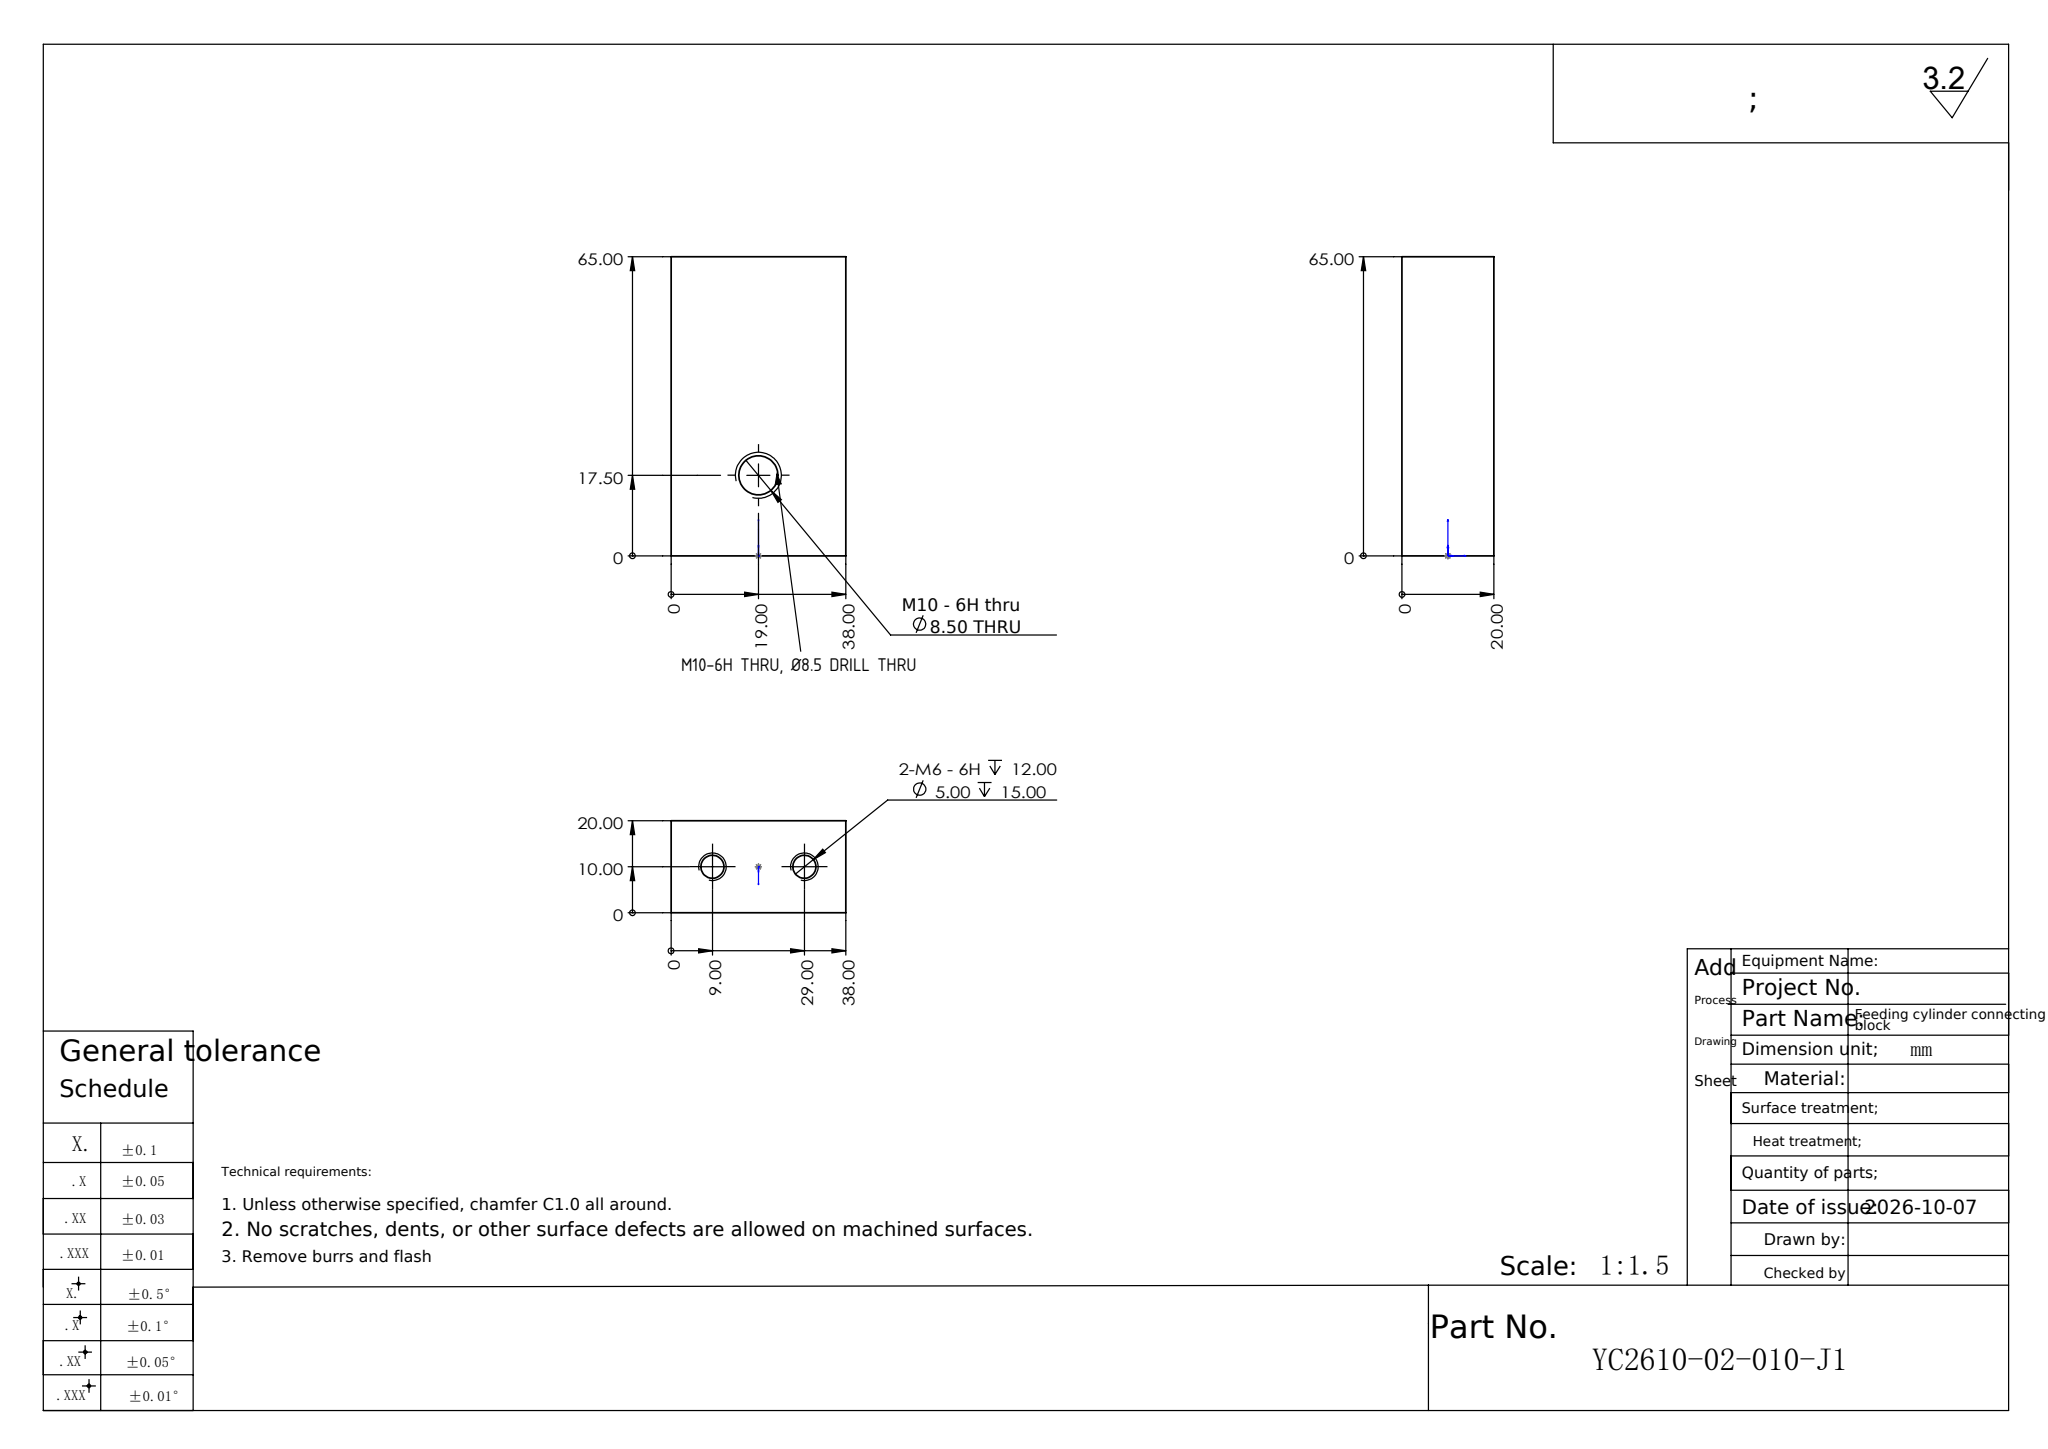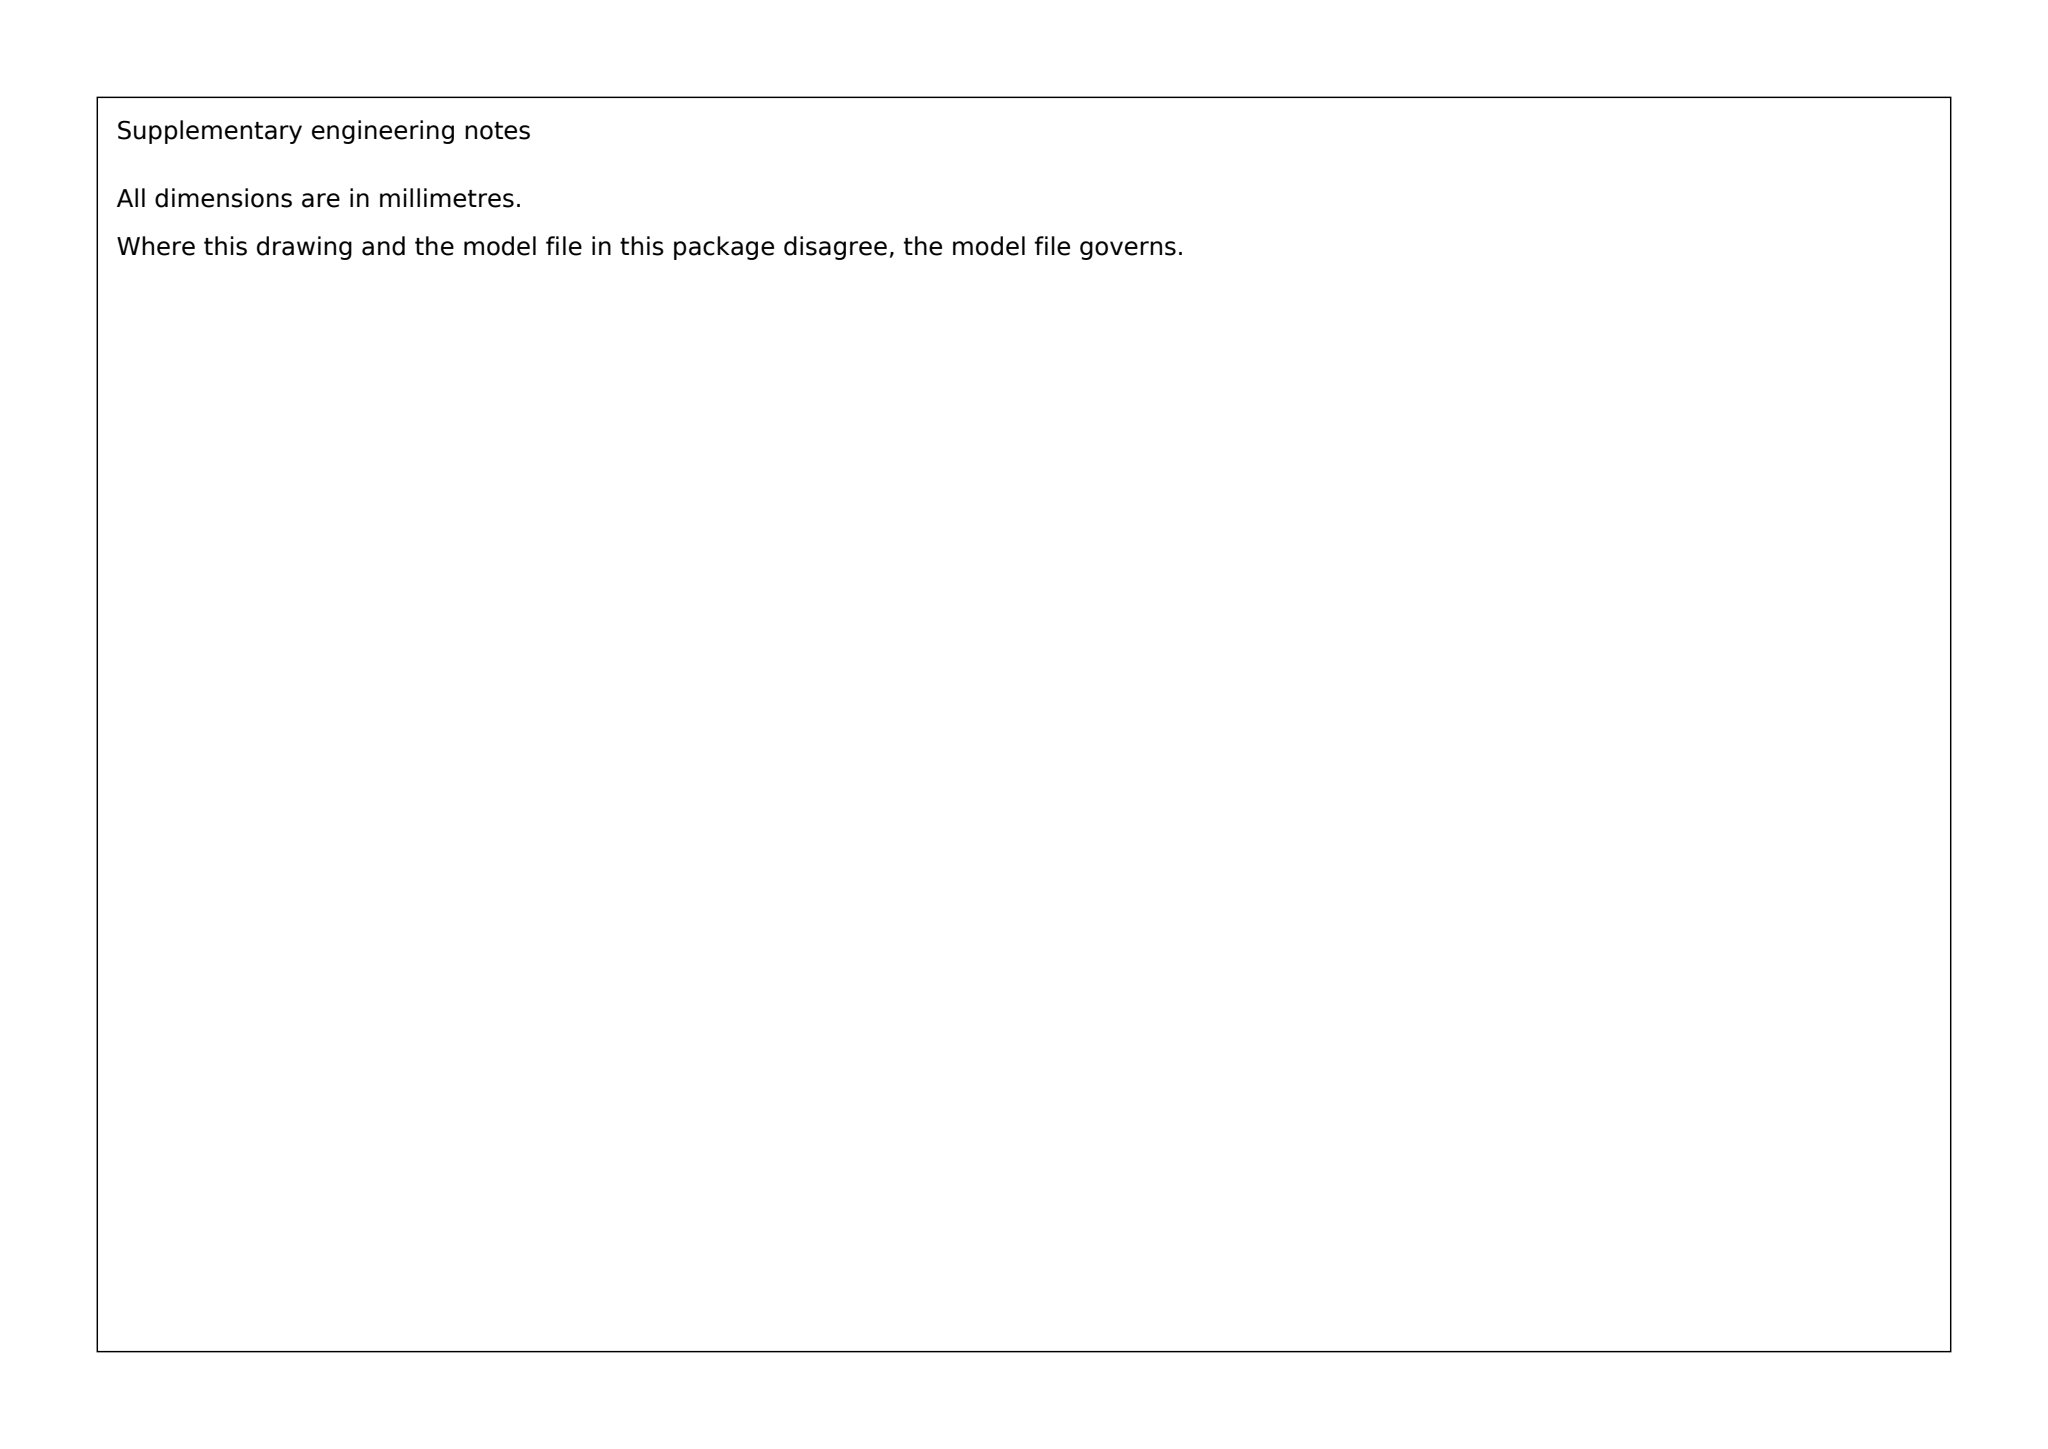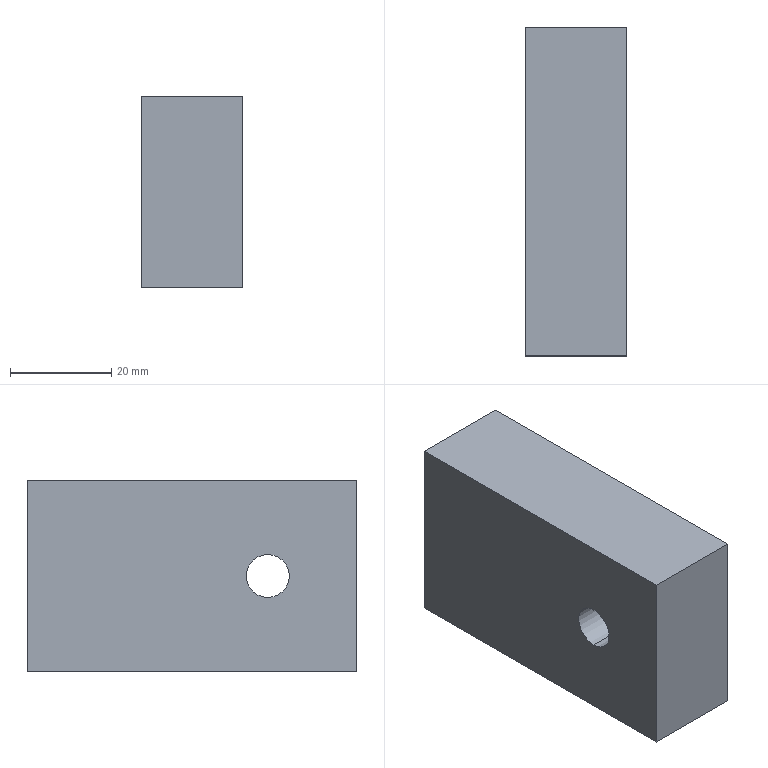Part | SolidWorks | mm | 1 solid | 16 faces | box 20 x 65 x 38 mm | volume 47656 mm3 | cylinder 6 | plane 6 | cone 4 | commonest cylinder face diameters 5 x4 8.5 x2
Drawing notes:
M10-6H THRU, Ø8.5 DRILL THRU 20 THK | from the solid: cylinder dia 8.5 axis x, length 20.0 = full x extent (planes x=0, x=20)
build123d program:
from build123d import *

# Parameters (mm, degrees)
SKETCH1_W             = 20
SKETCH1_H             = 38
BOSS_EXTRUDE1_DEPTH   = 65
M6_TAPPED_HOLE1_D     = 5
M6_TAPPED_HOLE1_DEPTH = 15
M6_TAPPED_HOLE1_TIP   = 1.502
M10_TAPPED_HOLE1_D    = 8.5


with BuildPart() as part:
    # Sketch1 → Boss-Extrude1 (new body)
    with BuildSketch(Plane(origin=(0, 0, 0), x_dir=(1, 0, 0), z_dir=(0, 1, 0))):
        Rectangle(SKETCH1_W, SKETCH1_H)
    extrude(amount=BOSS_EXTRUDE1_DEPTH)

    # M6 Tapped Hole1
    with Locations(Plane(origin=(0, 65, 0), x_dir=(1, 0, 0), z_dir=(0, 1, 0))):
        with Locations((0, 10), (0, -10)):
            Hole(M6_TAPPED_HOLE1_D / 2, depth=M6_TAPPED_HOLE1_DEPTH)
            with Locations((0, 0, -(M6_TAPPED_HOLE1_DEPTH + M6_TAPPED_HOLE1_TIP / 2))):  # 118° drill point
                Cone(0, M6_TAPPED_HOLE1_D / 2, M6_TAPPED_HOLE1_TIP, mode=Mode.SUBTRACT)

    # M10 Tapped Hole1 (through all)
    with Locations(Plane(origin=(10, 0, 0), x_dir=(0, 0, -1), z_dir=(1, 0, 0))):
        with Locations((0, 17.5)):
            Hole(M10_TAPPED_HOLE1_D / 2)


solid = part.part
STEP:
#1=CARTESIAN_POINT('',(-10.,17.5,4.25));
#2=VERTEX_POINT('',#1);
#3=CARTESIAN_POINT('',(-10.,17.5,-4.25));
#4=VERTEX_POINT('',#3);
#5=CARTESIAN_POINT('',(-10.,17.5,0.));
#6=DIRECTION('',(1.,0.,-0.));
#7=DIRECTION('',(0.,0.,-1.));
#8=AXIS2_PLACEMENT_3D('',#5,#6,#7);
#9=CIRCLE('',#8,4.25);
#10=EDGE_CURVE('',#2,#4,#9,.T.);
#11=ORIENTED_EDGE('',*,*,#10,.F.);
#12=CARTESIAN_POINT('',(10.,17.5,4.25));
#13=VERTEX_POINT('',#12);
#14=CARTESIAN_POINT('',(10.,17.5,4.25));
#15=DIRECTION('',(1.,0.,-0.));
#16=VECTOR('',#15,1000.);
#17=LINE('',#14,#16);
#18=EDGE_CURVE('',#2,#13,#17,.T.);
#19=ORIENTED_EDGE('',*,*,#18,.T.);
#20=CARTESIAN_POINT('',(10.,17.5,-4.25));
#21=VERTEX_POINT('',#20);
#22=CARTESIAN_POINT('',(10.,17.5,-0.));
#23=DIRECTION('',(1.,0.,-0.));
#24=DIRECTION('',(0.,0.,-1.));
#25=AXIS2_PLACEMENT_3D('',#22,#23,#24);
#26=CIRCLE('',#25,4.25);
#27=EDGE_CURVE('',#13,#21,#26,.T.);
#28=ORIENTED_EDGE('',*,*,#27,.T.);
#29=CARTESIAN_POINT('',(10.,17.5,-4.25));
#30=DIRECTION('',(1.,0.,-0.));
#31=VECTOR('',#30,1000.);
#32=LINE('',#29,#31);
#33=EDGE_CURVE('',#4,#21,#32,.T.);
#34=ORIENTED_EDGE('',*,*,#33,.F.);
#35=EDGE_LOOP('',(#11,#19,#28,#34));
#36=FACE_OUTER_BOUND('',#35,.T.);
#37=CARTESIAN_POINT('',(10.,17.5,-0.));
#38=DIRECTION('',(1.,0.,-0.));
#39=DIRECTION('',(0.,0.,-1.));
#40=AXIS2_PLACEMENT_3D('',#37,#38,#39);
#41=CYLINDRICAL_SURFACE('',#40,4.25);
#42=ADVANCED_FACE('',(#36),#41,.F.);
#43=CARTESIAN_POINT('',(0.,50.,-12.5));
#44=VERTEX_POINT('',#43);
#45=CARTESIAN_POINT('',(0.,50.,-7.5));
#46=VERTEX_POINT('',#45);
#47=CARTESIAN_POINT('',(0.,50.,-10.));
#48=DIRECTION('',(0.,1.,0.));
#49=DIRECTION('',(0.,0.,1.));
#50=AXIS2_PLACEMENT_3D('',#47,#48,#49);
#51=CIRCLE('',#50,2.5);
#52=EDGE_CURVE('',#44,#46,#51,.T.);
#53=ORIENTED_EDGE('',*,*,#52,.F.);
#54=CARTESIAN_POINT('',(0.,65.,-12.5));
#55=VERTEX_POINT('',#54);
#56=CARTESIAN_POINT('',(0.,65.,-12.5));
#57=DIRECTION('',(0.,1.,0.));
#58=VECTOR('',#57,1000.);
#59=LINE('',#56,#58);
#60=EDGE_CURVE('',#44,#55,#59,.T.);
#61=ORIENTED_EDGE('',*,*,#60,.T.);
#62=CARTESIAN_POINT('',(0.,65.,-7.5));
#63=VERTEX_POINT('',#62);
#64=CARTESIAN_POINT('',(0.,65.,-10.));
#65=DIRECTION('',(0.,1.,0.));
#66=DIRECTION('',(0.,0.,1.));
#67=AXIS2_PLACEMENT_3D('',#64,#65,#66);
#68=CIRCLE('',#67,2.5);
#69=EDGE_CURVE('',#55,#63,#68,.T.);
#70=ORIENTED_EDGE('',*,*,#69,.T.);
#71=CARTESIAN_POINT('',(0.,65.,-7.5));
#72=DIRECTION('',(0.,1.,0.));
#73=VECTOR('',#72,1000.);
#74=LINE('',#71,#73);
#75=EDGE_CURVE('',#46,#63,#74,.T.);
#76=ORIENTED_EDGE('',*,*,#75,.F.);
#77=EDGE_LOOP('',(#53,#61,#70,#76));
#78=FACE_OUTER_BOUND('',#77,.T.);
#79=CARTESIAN_POINT('',(0.,65.,-10.));
#80=DIRECTION('',(0.,1.,0.));
#81=DIRECTION('',(0.,0.,1.));
#82=AXIS2_PLACEMENT_3D('',#79,#80,#81);
#83=CYLINDRICAL_SURFACE('',#82,2.5);
#84=ADVANCED_FACE('',(#78),#83,.F.);
#85=CARTESIAN_POINT('',(-0.,48.498,-10.));
#86=VERTEX_POINT('',#85);
#87=CARTESIAN_POINT('',(0.,50.,-7.5));
#88=DIRECTION('',(0.,0.515,0.8572));
#89=VECTOR('',#88,1000.);
#90=LINE('',#87,#89);
#91=EDGE_CURVE('',#86,#46,#90,.T.);
#92=ORIENTED_EDGE('',*,*,#91,.F.);
#93=CARTESIAN_POINT('',(0.,50.,-12.5));
#94=DIRECTION('',(0.,0.515,-0.8572));
#95=VECTOR('',#94,1000.);
#96=LINE('',#93,#95);
#97=EDGE_CURVE('',#86,#44,#96,.T.);
#98=ORIENTED_EDGE('',*,*,#97,.T.);
#99=ORIENTED_EDGE('',*,*,#52,.T.);
#100=EDGE_LOOP('',(#92,#98,#99));
#101=FACE_OUTER_BOUND('',#100,.T.);
#102=CARTESIAN_POINT('',(0.,50.,-10.));
#103=DIRECTION('',(0.,1.,0.));
#104=DIRECTION('',(0.,0.,1.));
#105=AXIS2_PLACEMENT_3D('',#102,#103,#104);
#106=CONICAL_SURFACE('',#105,2.5,1.03);
#107=ADVANCED_FACE('',(#101),#106,.F.);
#108=CARTESIAN_POINT('',(0.,50.,7.5));
#109=VERTEX_POINT('',#108);
#110=CARTESIAN_POINT('',(0.,50.,12.5));
#111=VERTEX_POINT('',#110);
#112=CARTESIAN_POINT('',(0.,50.,10.));
#113=DIRECTION('',(0.,1.,0.));
#114=DIRECTION('',(0.,0.,1.));
#115=AXIS2_PLACEMENT_3D('',#112,#113,#114);
#116=CIRCLE('',#115,2.5);
#117=EDGE_CURVE('',#109,#111,#116,.T.);
#118=ORIENTED_EDGE('',*,*,#117,.F.);
#119=CARTESIAN_POINT('',(0.,65.,7.5));
#120=VERTEX_POINT('',#119);
#121=CARTESIAN_POINT('',(0.,65.,7.5));
#122=DIRECTION('',(0.,1.,0.));
#123=VECTOR('',#122,1000.);
#124=LINE('',#121,#123);
#125=EDGE_CURVE('',#109,#120,#124,.T.);
#126=ORIENTED_EDGE('',*,*,#125,.T.);
#127=CARTESIAN_POINT('',(0.,65.,12.5));
#128=VERTEX_POINT('',#127);
#129=CARTESIAN_POINT('',(0.,65.,10.));
#130=DIRECTION('',(0.,1.,0.));
#131=DIRECTION('',(0.,0.,1.));
#132=AXIS2_PLACEMENT_3D('',#129,#130,#131);
#133=CIRCLE('',#132,2.5);
#134=EDGE_CURVE('',#120,#128,#133,.T.);
#135=ORIENTED_EDGE('',*,*,#134,.T.);
#136=CARTESIAN_POINT('',(0.,65.,12.5));
#137=DIRECTION('',(0.,1.,0.));
#138=VECTOR('',#137,1000.);
#139=LINE('',#136,#138);
#140=EDGE_CURVE('',#111,#128,#139,.T.);
#141=ORIENTED_EDGE('',*,*,#140,.F.);
#142=EDGE_LOOP('',(#118,#126,#135,#141));
#143=FACE_OUTER_BOUND('',#142,.T.);
#144=CARTESIAN_POINT('',(0.,65.,10.));
#145=DIRECTION('',(0.,1.,0.));
#146=DIRECTION('',(0.,0.,1.));
#147=AXIS2_PLACEMENT_3D('',#144,#145,#146);
#148=CYLINDRICAL_SURFACE('',#147,2.5);
#149=ADVANCED_FACE('',(#143),#148,.F.);
#150=CARTESIAN_POINT('',(-0.,48.498,10.));
#151=VERTEX_POINT('',#150);
#152=CARTESIAN_POINT('',(0.,50.,12.5));
#153=DIRECTION('',(0.,0.515,0.8572));
#154=VECTOR('',#153,1000.);
#155=LINE('',#152,#154);
#156=EDGE_CURVE('',#151,#111,#155,.T.);
#157=ORIENTED_EDGE('',*,*,#156,.F.);
#158=CARTESIAN_POINT('',(0.,50.,7.5));
#159=DIRECTION('',(0.,0.515,-0.8572));
#160=VECTOR('',#159,1000.);
#161=LINE('',#158,#160);
#162=EDGE_CURVE('',#151,#109,#161,.T.);
#163=ORIENTED_EDGE('',*,*,#162,.T.);
#164=ORIENTED_EDGE('',*,*,#117,.T.);
#165=EDGE_LOOP('',(#157,#163,#164));
#166=FACE_OUTER_BOUND('',#165,.T.);
#167=CARTESIAN_POINT('',(0.,50.,10.));
#168=DIRECTION('',(0.,1.,0.));
#169=DIRECTION('',(0.,0.,1.));
#170=AXIS2_PLACEMENT_3D('',#167,#168,#169);
#171=CONICAL_SURFACE('',#170,2.5,1.03);
#172=ADVANCED_FACE('',(#166),#171,.F.);
#173=CARTESIAN_POINT('',(-10.,17.5,0.));
#174=DIRECTION('',(1.,0.,-0.));
#175=DIRECTION('',(0.,0.,-1.));
#176=AXIS2_PLACEMENT_3D('',#173,#174,#175);
#177=CIRCLE('',#176,4.25);
#178=EDGE_CURVE('',#4,#2,#177,.T.);
#179=ORIENTED_EDGE('',*,*,#178,.T.);
#180=ORIENTED_EDGE('',*,*,#10,.T.);
#181=EDGE_LOOP('',(#179,#180));
#182=FACE_BOUND('',#181,.T.);
#183=CARTESIAN_POINT('',(-10.,0.,-19.));
#184=VERTEX_POINT('',#183);
#185=CARTESIAN_POINT('',(-10.,0.,19.));
#186=VERTEX_POINT('',#185);
#187=CARTESIAN_POINT('',(-10.,0.,-19.));
#188=DIRECTION('',(0.,0.,1.));
#189=VECTOR('',#188,1000.);
#190=LINE('',#187,#189);
#191=EDGE_CURVE('',#184,#186,#190,.T.);
#192=ORIENTED_EDGE('',*,*,#191,.T.);
#193=CARTESIAN_POINT('',(-10.,65.,19.));
#194=VERTEX_POINT('',#193);
#195=CARTESIAN_POINT('',(-10.,65.,19.));
#196=DIRECTION('',(0.,-1.,0.));
#197=VECTOR('',#196,1000.);
#198=LINE('',#195,#197);
#199=EDGE_CURVE('',#194,#186,#198,.T.);
#200=ORIENTED_EDGE('',*,*,#199,.F.);
#201=CARTESIAN_POINT('',(-10.,65.,-19.));
#202=VERTEX_POINT('',#201);
#203=CARTESIAN_POINT('',(-10.,65.,-19.));
#204=DIRECTION('',(0.,0.,1.));
#205=VECTOR('',#204,1000.);
#206=LINE('',#203,#205);
#207=EDGE_CURVE('',#202,#194,#206,.T.);
#208=ORIENTED_EDGE('',*,*,#207,.F.);
#209=CARTESIAN_POINT('',(-10.,65.,-19.));
#210=DIRECTION('',(0.,-1.,0.));
#211=VECTOR('',#210,1000.);
#212=LINE('',#209,#211);
#213=EDGE_CURVE('',#202,#184,#212,.T.);
#214=ORIENTED_EDGE('',*,*,#213,.T.);
#215=EDGE_LOOP('',(#192,#200,#208,#214));
#216=FACE_OUTER_BOUND('',#215,.T.);
#217=CARTESIAN_POINT('',(-10.,65.,-19.));
#218=DIRECTION('',(1.,0.,-0.));
#219=DIRECTION('',(-0.,0.,-1.));
#220=AXIS2_PLACEMENT_3D('',#217,#218,#219);
#221=PLANE('',#220);
#222=ADVANCED_FACE('',(#182,#216),#221,.F.);
#223=CARTESIAN_POINT('',(10.,0.,19.));
#224=VERTEX_POINT('',#223);
#225=CARTESIAN_POINT('',(-10.,0.,19.));
#226=DIRECTION('',(1.,0.,0.));
#227=VECTOR('',#226,1000.);
#228=LINE('',#225,#227);
#229=EDGE_CURVE('',#186,#224,#228,.T.);
#230=ORIENTED_EDGE('',*,*,#229,.T.);
#231=CARTESIAN_POINT('',(10.,65.,19.));
#232=VERTEX_POINT('',#231);
#233=CARTESIAN_POINT('',(10.,65.,19.));
#234=DIRECTION('',(0.,-1.,0.));
#235=VECTOR('',#234,1000.);
#236=LINE('',#233,#235);
#237=EDGE_CURVE('',#232,#224,#236,.T.);
#238=ORIENTED_EDGE('',*,*,#237,.F.);
#239=CARTESIAN_POINT('',(-10.,65.,19.));
#240=DIRECTION('',(1.,0.,0.));
#241=VECTOR('',#240,1000.);
#242=LINE('',#239,#241);
#243=EDGE_CURVE('',#194,#232,#242,.T.);
#244=ORIENTED_EDGE('',*,*,#243,.F.);
#245=ORIENTED_EDGE('',*,*,#199,.T.);
#246=EDGE_LOOP('',(#230,#238,#244,#245));
#247=FACE_OUTER_BOUND('',#246,.T.);
#248=CARTESIAN_POINT('',(-10.,65.,19.));
#249=DIRECTION('',(0.,0.,-1.));
#250=DIRECTION('',(-1.,0.,0.));
#251=AXIS2_PLACEMENT_3D('',#248,#249,#250);
#252=PLANE('',#251);
#253=ADVANCED_FACE('',(#247),#252,.F.);
#254=CARTESIAN_POINT('',(10.,17.5,-0.));
#255=DIRECTION('',(1.,0.,-0.));
#256=DIRECTION('',(0.,0.,-1.));
#257=AXIS2_PLACEMENT_3D('',#254,#255,#256);
#258=CIRCLE('',#257,4.25);
#259=EDGE_CURVE('',#21,#13,#258,.T.);
#260=ORIENTED_EDGE('',*,*,#259,.F.);
#261=ORIENTED_EDGE('',*,*,#27,.F.);
#262=EDGE_LOOP('',(#260,#261));
#263=FACE_BOUND('',#262,.T.);
#264=CARTESIAN_POINT('',(10.,0.,-19.));
#265=VERTEX_POINT('',#264);
#266=CARTESIAN_POINT('',(10.,0.,-19.));
#267=DIRECTION('',(-0.,0.,-1.));
#268=VECTOR('',#267,1000.);
#269=LINE('',#266,#268);
#270=EDGE_CURVE('',#224,#265,#269,.T.);
#271=ORIENTED_EDGE('',*,*,#270,.T.);
#272=CARTESIAN_POINT('',(10.,65.,-19.));
#273=VERTEX_POINT('',#272);
#274=CARTESIAN_POINT('',(10.,65.,-19.));
#275=DIRECTION('',(0.,-1.,0.));
#276=VECTOR('',#275,1000.);
#277=LINE('',#274,#276);
#278=EDGE_CURVE('',#273,#265,#277,.T.);
#279=ORIENTED_EDGE('',*,*,#278,.F.);
#280=CARTESIAN_POINT('',(10.,65.,-19.));
#281=DIRECTION('',(-0.,0.,-1.));
#282=VECTOR('',#281,1000.);
#283=LINE('',#280,#282);
#284=EDGE_CURVE('',#232,#273,#283,.T.);
#285=ORIENTED_EDGE('',*,*,#284,.F.);
#286=ORIENTED_EDGE('',*,*,#237,.T.);
#287=EDGE_LOOP('',(#271,#279,#285,#286));
#288=FACE_OUTER_BOUND('',#287,.T.);
#289=CARTESIAN_POINT('',(10.,65.,-19.));
#290=DIRECTION('',(-1.,0.,0.));
#291=DIRECTION('',(0.,0.,1.));
#292=AXIS2_PLACEMENT_3D('',#289,#290,#291);
#293=PLANE('',#292);
#294=ADVANCED_FACE('',(#263,#288),#293,.F.);
#295=CARTESIAN_POINT('',(-10.,0.,-19.));
#296=DIRECTION('',(-1.,0.,0.));
#297=VECTOR('',#296,1000.);
#298=LINE('',#295,#297);
#299=EDGE_CURVE('',#265,#184,#298,.T.);
#300=ORIENTED_EDGE('',*,*,#299,.T.);
#301=ORIENTED_EDGE('',*,*,#213,.F.);
#302=CARTESIAN_POINT('',(-10.,65.,-19.));
#303=DIRECTION('',(-1.,0.,0.));
#304=VECTOR('',#303,1000.);
#305=LINE('',#302,#304);
#306=EDGE_CURVE('',#273,#202,#305,.T.);
#307=ORIENTED_EDGE('',*,*,#306,.F.);
#308=ORIENTED_EDGE('',*,*,#278,.T.);
#309=EDGE_LOOP('',(#300,#301,#307,#308));
#310=FACE_OUTER_BOUND('',#309,.T.);
#311=CARTESIAN_POINT('',(-10.,65.,-19.));
#312=DIRECTION('',(0.,0.,1.));
#313=DIRECTION('',(1.,0.,0.));
#314=AXIS2_PLACEMENT_3D('',#311,#312,#313);
#315=PLANE('',#314);
#316=ADVANCED_FACE('',(#310),#315,.F.);
#317=CARTESIAN_POINT('',(0.,65.,-10.));
#318=DIRECTION('',(0.,1.,0.));
#319=DIRECTION('',(0.,0.,1.));
#320=AXIS2_PLACEMENT_3D('',#317,#318,#319);
#321=CIRCLE('',#320,2.5);
#322=EDGE_CURVE('',#63,#55,#321,.T.);
#323=ORIENTED_EDGE('',*,*,#322,.F.);
#324=ORIENTED_EDGE('',*,*,#69,.F.);
#325=EDGE_LOOP('',(#323,#324));
#326=FACE_BOUND('',#325,.T.);
#327=CARTESIAN_POINT('',(0.,65.,10.));
#328=DIRECTION('',(0.,1.,0.));
#329=DIRECTION('',(0.,0.,1.));
#330=AXIS2_PLACEMENT_3D('',#327,#328,#329);
#331=CIRCLE('',#330,2.5);
#332=EDGE_CURVE('',#128,#120,#331,.T.);
#333=ORIENTED_EDGE('',*,*,#332,.F.);
#334=ORIENTED_EDGE('',*,*,#134,.F.);
#335=EDGE_LOOP('',(#333,#334));
#336=FACE_BOUND('',#335,.T.);
#337=ORIENTED_EDGE('',*,*,#207,.T.);
#338=ORIENTED_EDGE('',*,*,#243,.T.);
#339=ORIENTED_EDGE('',*,*,#284,.T.);
#340=ORIENTED_EDGE('',*,*,#306,.T.);
#341=EDGE_LOOP('',(#337,#338,#339,#340));
#342=FACE_OUTER_BOUND('',#341,.T.);
#343=CARTESIAN_POINT('',(0.,65.,0.));
#344=DIRECTION('',(0.,1.,0.));
#345=DIRECTION('',(0.,0.,1.));
#346=AXIS2_PLACEMENT_3D('',#343,#344,#345);
#347=PLANE('',#346);
#348=ADVANCED_FACE('',(#326,#336,#342),#347,.T.);
#349=ORIENTED_EDGE('',*,*,#191,.F.);
#350=ORIENTED_EDGE('',*,*,#299,.F.);
#351=ORIENTED_EDGE('',*,*,#270,.F.);
#352=ORIENTED_EDGE('',*,*,#229,.F.);
#353=EDGE_LOOP('',(#349,#350,#351,#352));
#354=FACE_OUTER_BOUND('',#353,.T.);
#355=CARTESIAN_POINT('',(0.,0.,0.));
#356=DIRECTION('',(0.,1.,0.));
#357=DIRECTION('',(0.,0.,1.));
#358=AXIS2_PLACEMENT_3D('',#355,#356,#357);
#359=PLANE('',#358);
#360=ADVANCED_FACE('',(#354),#359,.F.);
#361=ORIENTED_EDGE('',*,*,#162,.F.);
#362=ORIENTED_EDGE('',*,*,#156,.T.);
#363=CARTESIAN_POINT('',(0.,50.,10.));
#364=DIRECTION('',(0.,1.,0.));
#365=DIRECTION('',(0.,0.,1.));
#366=AXIS2_PLACEMENT_3D('',#363,#364,#365);
#367=CIRCLE('',#366,2.5);
#368=EDGE_CURVE('',#111,#109,#367,.T.);
#369=ORIENTED_EDGE('',*,*,#368,.T.);
#370=EDGE_LOOP('',(#361,#362,#369));
#371=FACE_OUTER_BOUND('',#370,.T.);
#372=CARTESIAN_POINT('',(0.,50.,10.));
#373=DIRECTION('',(0.,1.,0.));
#374=DIRECTION('',(0.,0.,1.));
#375=AXIS2_PLACEMENT_3D('',#372,#373,#374);
#376=CONICAL_SURFACE('',#375,2.5,1.03);
#377=ADVANCED_FACE('',(#371),#376,.F.);
#378=ORIENTED_EDGE('',*,*,#125,.F.);
#379=ORIENTED_EDGE('',*,*,#368,.F.);
#380=ORIENTED_EDGE('',*,*,#140,.T.);
#381=ORIENTED_EDGE('',*,*,#332,.T.);
#382=EDGE_LOOP('',(#378,#379,#380,#381));
#383=FACE_OUTER_BOUND('',#382,.T.);
#384=CARTESIAN_POINT('',(0.,65.,10.));
#385=DIRECTION('',(0.,1.,0.));
#386=DIRECTION('',(0.,0.,1.));
#387=AXIS2_PLACEMENT_3D('',#384,#385,#386);
#388=CYLINDRICAL_SURFACE('',#387,2.5);
#389=ADVANCED_FACE('',(#383),#388,.F.);
#390=ORIENTED_EDGE('',*,*,#97,.F.);
#391=ORIENTED_EDGE('',*,*,#91,.T.);
#392=CARTESIAN_POINT('',(0.,50.,-10.));
#393=DIRECTION('',(0.,1.,0.));
#394=DIRECTION('',(0.,0.,1.));
#395=AXIS2_PLACEMENT_3D('',#392,#393,#394);
#396=CIRCLE('',#395,2.5);
#397=EDGE_CURVE('',#46,#44,#396,.T.);
#398=ORIENTED_EDGE('',*,*,#397,.T.);
#399=EDGE_LOOP('',(#390,#391,#398));
#400=FACE_OUTER_BOUND('',#399,.T.);
#401=CARTESIAN_POINT('',(0.,50.,-10.));
#402=DIRECTION('',(0.,1.,0.));
#403=DIRECTION('',(0.,0.,1.));
#404=AXIS2_PLACEMENT_3D('',#401,#402,#403);
#405=CONICAL_SURFACE('',#404,2.5,1.03);
#406=ADVANCED_FACE('',(#400),#405,.F.);
#407=ORIENTED_EDGE('',*,*,#60,.F.);
#408=ORIENTED_EDGE('',*,*,#397,.F.);
#409=ORIENTED_EDGE('',*,*,#75,.T.);
#410=ORIENTED_EDGE('',*,*,#322,.T.);
#411=EDGE_LOOP('',(#407,#408,#409,#410));
#412=FACE_OUTER_BOUND('',#411,.T.);
#413=CARTESIAN_POINT('',(0.,65.,-10.));
#414=DIRECTION('',(0.,1.,0.));
#415=DIRECTION('',(0.,0.,1.));
#416=AXIS2_PLACEMENT_3D('',#413,#414,#415);
#417=CYLINDRICAL_SURFACE('',#416,2.5);
#418=ADVANCED_FACE('',(#412),#417,.F.);
#419=ORIENTED_EDGE('',*,*,#18,.F.);
#420=ORIENTED_EDGE('',*,*,#178,.F.);
#421=ORIENTED_EDGE('',*,*,#33,.T.);
#422=ORIENTED_EDGE('',*,*,#259,.T.);
#423=EDGE_LOOP('',(#419,#420,#421,#422));
#424=FACE_OUTER_BOUND('',#423,.T.);
#425=CARTESIAN_POINT('',(10.,17.5,-0.));
#426=DIRECTION('',(1.,0.,-0.));
#427=DIRECTION('',(0.,0.,-1.));
#428=AXIS2_PLACEMENT_3D('',#425,#426,#427);
#429=CYLINDRICAL_SURFACE('',#428,4.25);
#430=ADVANCED_FACE('',(#424),#429,.F.);
#431=CLOSED_SHELL('',(#42,#84,#107,#149,#172,#222,#253,#294,#316,#348,#360,#377,#389,#406,#418,#430));
#432=MANIFOLD_SOLID_BREP('',#431);
#433=CARTESIAN_POINT('',(0.,0.,0.));
#434=DIRECTION('',(0.,0.,1.));
#435=DIRECTION('',(1.,0.,0.));
#436=AXIS2_PLACEMENT_3D('',#433,#434,#435);
#437=(LENGTH_UNIT()NAMED_UNIT(*)SI_UNIT(.MILLI.,.METRE.));
#438=UNCERTAINTY_MEASURE_WITH_UNIT(LENGTH_MEASURE(0.00001),#437,'','');
#439=(NAMED_UNIT(*)PLANE_ANGLE_UNIT()SI_UNIT($,.RADIAN.));
#440=(NAMED_UNIT(*)SI_UNIT($,.STERADIAN.)SOLID_ANGLE_UNIT());
#441=(GEOMETRIC_REPRESENTATION_CONTEXT(3)GLOBAL_UNCERTAINTY_ASSIGNED_CONTEXT((#438))GLOBAL_UNIT_ASSIGNED_CONTEXT((#437,#439,#440))REPRESENTATION_CONTEXT('',''));
#442=ADVANCED_BREP_SHAPE_REPRESENTATION('',(#432,#436),#441);